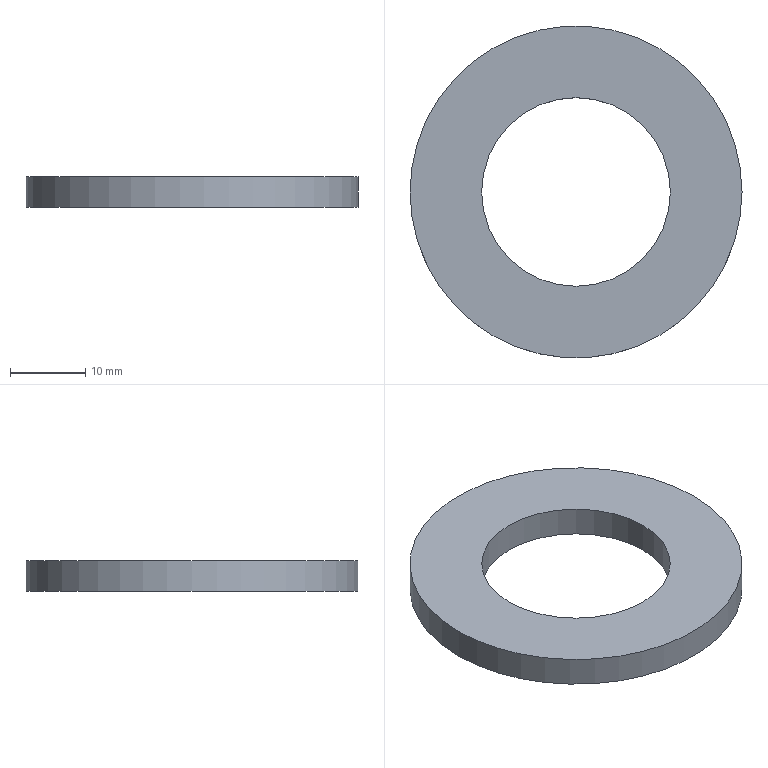Component | NX | GB-T97_1-2002_M24_2 | 1 solid | 4 faces | box 44 x 44 x 4 mm | volume 4119 mm3 | cylinder 2 | plane 2 | commonest cylinder face diameters 44 x1 25 x1
STEP:
#1=CARTESIAN_POINT('',(0.,0.,0.));
#2=DIRECTION('',(0.,0.,1.));
#3=DIRECTION('',(1.,0.,0.));
#4=AXIS2_PLACEMENT_3D('',#1,#2,#3);
#5=CARTESIAN_POINT('',(148.,-80.,50.));
#6=VERTEX_POINT('',#5);
#7=CARTESIAN_POINT('',(170.,-80.,50.));
#8=DIRECTION('',(0.,0.,-1.));
#9=DIRECTION('',(-1.,0.,0.));
#10=AXIS2_PLACEMENT_3D('',#7,#8,#9);
#11=CIRCLE('',#10,22.);
#12=CARTESIAN_POINT('',(170.,-80.,50.));
#13=DIRECTION('',(0.,0.,1.));
#14=DIRECTION('',(1.,0.,0.));
#15=AXIS2_PLACEMENT_3D('',#12,#13,#14);
#16=CYLINDRICAL_SURFACE('',#15,22.);
#17=CARTESIAN_POINT('',(9.425,0.));
#18=DIRECTION('',(-1.,0.));
#19=VECTOR('',#18,1.);
#20=LINE('',#17,#19);
#21=(GEOMETRIC_REPRESENTATION_CONTEXT(2)PARAMETRIC_REPRESENTATION_CONTEXT()REPRESENTATION_CONTEXT('',''));
#22=DEFINITIONAL_REPRESENTATION('',(#20),#21);
#23=PCURVE('',#16,#22);
#24=CARTESIAN_POINT('',(170.,-80.,50.));
#25=DIRECTION('',(0.,0.,-1.));
#26=DIRECTION('',(-1.,0.,0.));
#27=AXIS2_PLACEMENT_3D('',#24,#25,#26);
#28=PLANE('',#27);
#29=CARTESIAN_POINT('',(0.,0.));
#30=DIRECTION('',(1.,0.));
#31=AXIS2_PLACEMENT_2D('',#29,#30);
#32=CIRCLE('',#31,22.);
#33=(GEOMETRIC_REPRESENTATION_CONTEXT(2)PARAMETRIC_REPRESENTATION_CONTEXT()REPRESENTATION_CONTEXT('',''));
#34=DEFINITIONAL_REPRESENTATION('',(#32),#33);
#35=PCURVE('',#28,#34);
#36=SURFACE_CURVE('',#11,(#23,#35),.PCURVE_S1.);
#37=EDGE_CURVE('',#6,#6,#36,.T.);
#38=ORIENTED_EDGE('',*,*,#37,.F.);
#39=CARTESIAN_POINT('',(148.,-80.,54.));
#40=VERTEX_POINT('',#39);
#41=CARTESIAN_POINT('',(148.,-80.,50.));
#42=CARTESIAN_POINT('',(148.,-80.,54.));
#43=B_SPLINE_CURVE_WITH_KNOTS('',1,(#41,#42),.UNSPECIFIED.,.F.,.F.,(2,2),(0.,4.),.PIECEWISE_BEZIER_KNOTS.);
#44=CARTESIAN_POINT('',(9.425,0.));
#45=DIRECTION('',(0.,1.));
#46=VECTOR('',#45,1.);
#47=LINE('',#44,#46);
#48=(GEOMETRIC_REPRESENTATION_CONTEXT(2)PARAMETRIC_REPRESENTATION_CONTEXT()REPRESENTATION_CONTEXT('',''));
#49=DEFINITIONAL_REPRESENTATION('',(#47),#48);
#50=PCURVE('',#16,#49);
#51=CARTESIAN_POINT('',(3.142,0.));
#52=DIRECTION('',(0.,1.));
#53=VECTOR('',#52,1.);
#54=LINE('',#51,#53);
#55=(GEOMETRIC_REPRESENTATION_CONTEXT(2)PARAMETRIC_REPRESENTATION_CONTEXT()REPRESENTATION_CONTEXT('',''));
#56=DEFINITIONAL_REPRESENTATION('',(#54),#55);
#57=PCURVE('',#16,#56);
#58=SEAM_CURVE('',#43,(#50,#57),.PCURVE_S1.);
#59=EDGE_CURVE('',#6,#40,#58,.T.);
#60=ORIENTED_EDGE('',*,*,#59,.T.);
#61=CARTESIAN_POINT('',(170.,-80.,54.));
#62=DIRECTION('',(0.,0.,-1.));
#63=DIRECTION('',(-1.,0.,0.));
#64=AXIS2_PLACEMENT_3D('',#61,#62,#63);
#65=CIRCLE('',#64,22.);
#66=CARTESIAN_POINT('',(9.425,4.));
#67=DIRECTION('',(-1.,0.));
#68=VECTOR('',#67,1.);
#69=LINE('',#66,#68);
#70=(GEOMETRIC_REPRESENTATION_CONTEXT(2)PARAMETRIC_REPRESENTATION_CONTEXT()REPRESENTATION_CONTEXT('',''));
#71=DEFINITIONAL_REPRESENTATION('',(#69),#70);
#72=PCURVE('',#16,#71);
#73=CARTESIAN_POINT('',(170.,-80.,54.));
#74=DIRECTION('',(0.,0.,-1.));
#75=DIRECTION('',(-1.,0.,0.));
#76=AXIS2_PLACEMENT_3D('',#73,#74,#75);
#77=PLANE('',#76);
#78=CARTESIAN_POINT('',(0.,0.));
#79=DIRECTION('',(1.,0.));
#80=AXIS2_PLACEMENT_2D('',#78,#79);
#81=CIRCLE('',#80,22.);
#82=(GEOMETRIC_REPRESENTATION_CONTEXT(2)PARAMETRIC_REPRESENTATION_CONTEXT()REPRESENTATION_CONTEXT('',''));
#83=DEFINITIONAL_REPRESENTATION('',(#81),#82);
#84=PCURVE('',#77,#83);
#85=SURFACE_CURVE('',#65,(#72,#84),.PCURVE_S1.);
#86=EDGE_CURVE('',#40,#40,#85,.T.);
#87=ORIENTED_EDGE('',*,*,#86,.T.);
#88=ORIENTED_EDGE('',*,*,#59,.F.);
#89=EDGE_LOOP('',(#38,#60,#87,#88));
#90=FACE_BOUND('',#89,.T.);
#91=ADVANCED_FACE('',(#90),#16,.T.);
#92=CARTESIAN_POINT('',(157.5,-80.,50.));
#93=VERTEX_POINT('',#92);
#94=CARTESIAN_POINT('',(170.,-80.,50.));
#95=DIRECTION('',(0.,0.,-1.));
#96=DIRECTION('',(-1.,0.,0.));
#97=AXIS2_PLACEMENT_3D('',#94,#95,#96);
#98=CIRCLE('',#97,12.5);
#99=CARTESIAN_POINT('',(170.,-80.,50.));
#100=DIRECTION('',(0.,0.,1.));
#101=DIRECTION('',(1.,0.,0.));
#102=AXIS2_PLACEMENT_3D('',#99,#100,#101);
#103=CYLINDRICAL_SURFACE('',#102,12.5);
#104=CARTESIAN_POINT('',(9.425,0.));
#105=DIRECTION('',(-1.,0.));
#106=VECTOR('',#105,1.);
#107=LINE('',#104,#106);
#108=(GEOMETRIC_REPRESENTATION_CONTEXT(2)PARAMETRIC_REPRESENTATION_CONTEXT()REPRESENTATION_CONTEXT('',''));
#109=DEFINITIONAL_REPRESENTATION('',(#107),#108);
#110=PCURVE('',#103,#109);
#111=CARTESIAN_POINT('',(0.,0.));
#112=DIRECTION('',(1.,0.));
#113=AXIS2_PLACEMENT_2D('',#111,#112);
#114=CIRCLE('',#113,12.5);
#115=(GEOMETRIC_REPRESENTATION_CONTEXT(2)PARAMETRIC_REPRESENTATION_CONTEXT()REPRESENTATION_CONTEXT('',''));
#116=DEFINITIONAL_REPRESENTATION('',(#114),#115);
#117=PCURVE('',#28,#116);
#118=SURFACE_CURVE('',#98,(#110,#117),.PCURVE_S1.);
#119=EDGE_CURVE('',#93,#93,#118,.T.);
#120=ORIENTED_EDGE('',*,*,#119,.F.);
#121=CARTESIAN_POINT('',(157.5,-80.,54.));
#122=VERTEX_POINT('',#121);
#123=CARTESIAN_POINT('',(157.5,-80.,50.));
#124=CARTESIAN_POINT('',(157.5,-80.,54.));
#125=B_SPLINE_CURVE_WITH_KNOTS('',1,(#123,#124),.UNSPECIFIED.,.F.,.F.,(2,2),(0.,4.),.PIECEWISE_BEZIER_KNOTS.);
#126=CARTESIAN_POINT('',(9.425,0.));
#127=DIRECTION('',(0.,1.));
#128=VECTOR('',#127,1.);
#129=LINE('',#126,#128);
#130=(GEOMETRIC_REPRESENTATION_CONTEXT(2)PARAMETRIC_REPRESENTATION_CONTEXT()REPRESENTATION_CONTEXT('',''));
#131=DEFINITIONAL_REPRESENTATION('',(#129),#130);
#132=PCURVE('',#103,#131);
#133=CARTESIAN_POINT('',(3.142,0.));
#134=DIRECTION('',(0.,1.));
#135=VECTOR('',#134,1.);
#136=LINE('',#133,#135);
#137=(GEOMETRIC_REPRESENTATION_CONTEXT(2)PARAMETRIC_REPRESENTATION_CONTEXT()REPRESENTATION_CONTEXT('',''));
#138=DEFINITIONAL_REPRESENTATION('',(#136),#137);
#139=PCURVE('',#103,#138);
#140=SEAM_CURVE('',#125,(#132,#139),.PCURVE_S1.);
#141=EDGE_CURVE('',#93,#122,#140,.T.);
#142=ORIENTED_EDGE('',*,*,#141,.T.);
#143=CARTESIAN_POINT('',(170.,-80.,54.));
#144=DIRECTION('',(0.,0.,-1.));
#145=DIRECTION('',(-1.,0.,0.));
#146=AXIS2_PLACEMENT_3D('',#143,#144,#145);
#147=CIRCLE('',#146,12.5);
#148=CARTESIAN_POINT('',(9.425,4.));
#149=DIRECTION('',(-1.,0.));
#150=VECTOR('',#149,1.);
#151=LINE('',#148,#150);
#152=(GEOMETRIC_REPRESENTATION_CONTEXT(2)PARAMETRIC_REPRESENTATION_CONTEXT()REPRESENTATION_CONTEXT('',''));
#153=DEFINITIONAL_REPRESENTATION('',(#151),#152);
#154=PCURVE('',#103,#153);
#155=CARTESIAN_POINT('',(0.,0.));
#156=DIRECTION('',(1.,0.));
#157=AXIS2_PLACEMENT_2D('',#155,#156);
#158=CIRCLE('',#157,12.5);
#159=(GEOMETRIC_REPRESENTATION_CONTEXT(2)PARAMETRIC_REPRESENTATION_CONTEXT()REPRESENTATION_CONTEXT('',''));
#160=DEFINITIONAL_REPRESENTATION('',(#158),#159);
#161=PCURVE('',#77,#160);
#162=SURFACE_CURVE('',#147,(#154,#161),.PCURVE_S1.);
#163=EDGE_CURVE('',#122,#122,#162,.T.);
#164=ORIENTED_EDGE('',*,*,#163,.T.);
#165=ORIENTED_EDGE('',*,*,#141,.F.);
#166=EDGE_LOOP('',(#120,#142,#164,#165));
#167=FACE_BOUND('',#166,.F.);
#168=ADVANCED_FACE('',(#167),#103,.F.);
#169=ORIENTED_EDGE('',*,*,#37,.T.);
#170=EDGE_LOOP('',(#169));
#171=FACE_BOUND('',#170,.T.);
#172=ORIENTED_EDGE('',*,*,#119,.F.);
#173=EDGE_LOOP('',(#172));
#174=FACE_BOUND('',#173,.T.);
#175=ADVANCED_FACE('',(#171,#174),#28,.T.);
#176=ORIENTED_EDGE('',*,*,#86,.F.);
#177=EDGE_LOOP('',(#176));
#178=FACE_BOUND('',#177,.T.);
#179=ORIENTED_EDGE('',*,*,#163,.T.);
#180=EDGE_LOOP('',(#179));
#181=FACE_BOUND('',#180,.T.);
#182=ADVANCED_FACE('',(#178,#181),#77,.F.);
#183=CLOSED_SHELL('',(#91,#168,#175,#182));
#184=MANIFOLD_SOLID_BREP('',#183);
#185=(LENGTH_UNIT()NAMED_UNIT(*)SI_UNIT(.MILLI.,.METRE.));
#186=UNCERTAINTY_MEASURE_WITH_UNIT(LENGTH_MEASURE(0.00001),#185,'','');
#187=(NAMED_UNIT(*)PLANE_ANGLE_UNIT()SI_UNIT($,.RADIAN.));
#188=(NAMED_UNIT(*)SI_UNIT($,.STERADIAN.)SOLID_ANGLE_UNIT());
#189=(GEOMETRIC_REPRESENTATION_CONTEXT(3)GLOBAL_UNCERTAINTY_ASSIGNED_CONTEXT((#186))GLOBAL_UNIT_ASSIGNED_CONTEXT((#185,#187,#188))REPRESENTATION_CONTEXT('',''));
#190=ADVANCED_BREP_SHAPE_REPRESENTATION('',(#4,#184),#189);